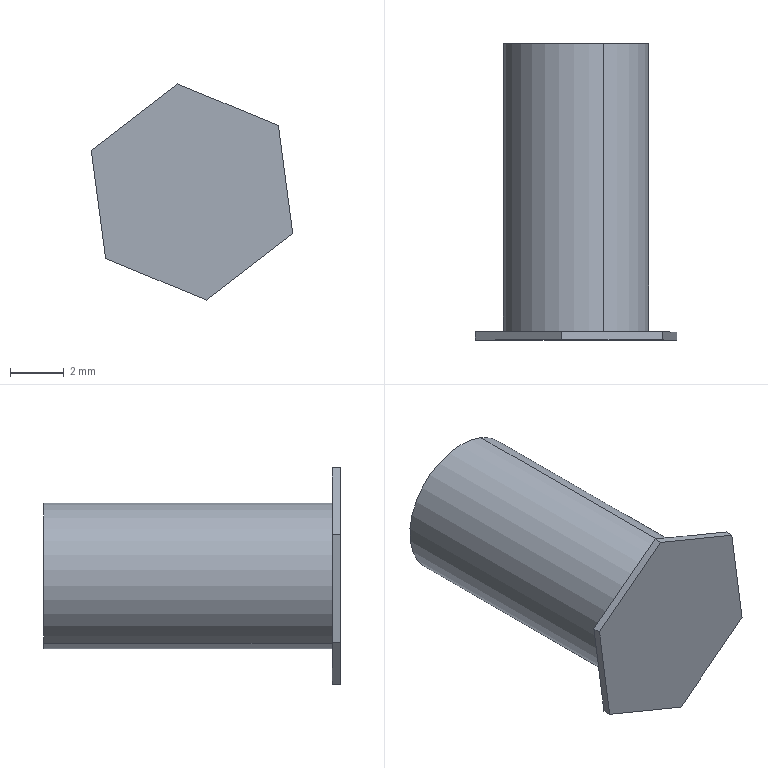Component | SolidWorks | P16BoxWeldment-1_BSO-M3-10-1 | 1 solid | 14 faces | box 7.48 x 11 x 8.02 mm | volume 201 mm3 | plane 10 | cylinder 4 | commonest cylinder face diameters 3 x2 5.4 x2
STEP:
#1=CARTESIAN_POINT('',(11.267,-9.398,0.4247));
#2=VERTEX_POINT('',#1);
#3=CARTESIAN_POINT('',(11.222,-9.398,0.3155));
#4=VERTEX_POINT('',#3);
#5=CARTESIAN_POINT('',(11.244,-9.398,0.3701));
#6=DIRECTION('',(-0.,1.,-0.));
#7=DIRECTION('',(-0.3816,0.,-0.9243));
#8=AXIS2_PLACEMENT_3D('',#5,#6,#7);
#9=CIRCLE('',#8,0.05906);
#10=EDGE_CURVE('',#2,#4,#9,.T.);
#11=ORIENTED_EDGE('',*,*,#10,.F.);
#12=CARTESIAN_POINT('',(11.267,-9.083,0.4247));
#13=VERTEX_POINT('',#12);
#14=CARTESIAN_POINT('',(11.267,-9.398,0.4247));
#15=DIRECTION('',(-0.,1.,-0.));
#16=VECTOR('',#15,39.37);
#17=LINE('',#14,#16);
#18=EDGE_CURVE('',#2,#13,#17,.T.);
#19=ORIENTED_EDGE('',*,*,#18,.T.);
#20=CARTESIAN_POINT('',(11.222,-9.083,0.3155));
#21=VERTEX_POINT('',#20);
#22=CARTESIAN_POINT('',(11.244,-9.083,0.3701));
#23=DIRECTION('',(-0.,1.,-0.));
#24=DIRECTION('',(-0.3816,0.,-0.9243));
#25=AXIS2_PLACEMENT_3D('',#22,#23,#24);
#26=CIRCLE('',#25,0.05906);
#27=EDGE_CURVE('',#13,#21,#26,.T.);
#28=ORIENTED_EDGE('',*,*,#27,.T.);
#29=CARTESIAN_POINT('',(11.222,-9.398,0.3155));
#30=DIRECTION('',(-0.,1.,-0.));
#31=VECTOR('',#30,39.37);
#32=LINE('',#29,#31);
#33=EDGE_CURVE('',#4,#21,#32,.T.);
#34=ORIENTED_EDGE('',*,*,#33,.F.);
#35=EDGE_LOOP('',(#11,#19,#28,#34));
#36=FACE_OUTER_BOUND('',#35,.T.);
#37=CARTESIAN_POINT('',(11.244,-9.398,0.3701));
#38=DIRECTION('',(-0.,1.,-0.));
#39=DIRECTION('',(-0.3816,0.,-0.9243));
#40=AXIS2_PLACEMENT_3D('',#37,#38,#39);
#41=CYLINDRICAL_SURFACE('',#40,0.05906);
#42=ADVANCED_FACE('',(#36),#41,.F.);
#43=CARTESIAN_POINT('',(11.204,-9.083,0.2718));
#44=VERTEX_POINT('',#43);
#45=CARTESIAN_POINT('',(11.285,-9.083,0.4683));
#46=VERTEX_POINT('',#45);
#47=CARTESIAN_POINT('',(11.244,-9.083,0.3701));
#48=DIRECTION('',(-0.,1.,-0.));
#49=DIRECTION('',(-0.3816,0.,-0.9243));
#50=AXIS2_PLACEMENT_3D('',#47,#48,#49);
#51=CIRCLE('',#50,0.1063);
#52=EDGE_CURVE('',#44,#46,#51,.T.);
#53=ORIENTED_EDGE('',*,*,#52,.F.);
#54=CARTESIAN_POINT('',(11.204,-9.504,0.2718));
#55=VERTEX_POINT('',#54);
#56=CARTESIAN_POINT('',(11.204,-9.083,0.2718));
#57=DIRECTION('',(0.,-1.,0.));
#58=VECTOR('',#57,39.37);
#59=LINE('',#56,#58);
#60=EDGE_CURVE('',#44,#55,#59,.T.);
#61=ORIENTED_EDGE('',*,*,#60,.T.);
#62=CARTESIAN_POINT('',(11.285,-9.504,0.4683));
#63=VERTEX_POINT('',#62);
#64=CARTESIAN_POINT('',(11.244,-9.504,0.3701));
#65=DIRECTION('',(0.,-1.,0.));
#66=DIRECTION('',(0.3816,0.,0.9243));
#67=AXIS2_PLACEMENT_3D('',#64,#65,#66);
#68=CIRCLE('',#67,0.1063);
#69=EDGE_CURVE('',#63,#55,#68,.T.);
#70=ORIENTED_EDGE('',*,*,#69,.F.);
#71=CARTESIAN_POINT('',(11.285,-9.083,0.4683));
#72=DIRECTION('',(0.,-1.,0.));
#73=VECTOR('',#72,39.37);
#74=LINE('',#71,#73);
#75=EDGE_CURVE('',#46,#63,#74,.T.);
#76=ORIENTED_EDGE('',*,*,#75,.F.);
#77=EDGE_LOOP('',(#53,#61,#70,#76));
#78=FACE_OUTER_BOUND('',#77,.T.);
#79=CARTESIAN_POINT('',(11.244,-9.083,0.3701));
#80=DIRECTION('',(0.,-1.,0.));
#81=DIRECTION('',(0.3816,0.,0.9243));
#82=AXIS2_PLACEMENT_3D('',#79,#80,#81);
#83=CYLINDRICAL_SURFACE('',#82,0.1063);
#84=ADVANCED_FACE('',(#78),#83,.T.);
#85=ORIENTED_EDGE('',*,*,#60,.F.);
#86=CARTESIAN_POINT('',(11.244,-9.083,0.3701));
#87=DIRECTION('',(-0.,1.,-0.));
#88=DIRECTION('',(-0.3816,0.,-0.9243));
#89=AXIS2_PLACEMENT_3D('',#86,#87,#88);
#90=CIRCLE('',#89,0.1063);
#91=EDGE_CURVE('',#46,#44,#90,.T.);
#92=ORIENTED_EDGE('',*,*,#91,.F.);
#93=ORIENTED_EDGE('',*,*,#75,.T.);
#94=CARTESIAN_POINT('',(11.244,-9.504,0.3701));
#95=DIRECTION('',(0.,-1.,0.));
#96=DIRECTION('',(0.3816,0.,0.9243));
#97=AXIS2_PLACEMENT_3D('',#94,#95,#96);
#98=CIRCLE('',#97,0.1063);
#99=EDGE_CURVE('',#55,#63,#98,.T.);
#100=ORIENTED_EDGE('',*,*,#99,.F.);
#101=EDGE_LOOP('',(#85,#92,#93,#100));
#102=FACE_OUTER_BOUND('',#101,.T.);
#103=CARTESIAN_POINT('',(11.244,-9.083,0.3701));
#104=DIRECTION('',(0.,-1.,0.));
#105=DIRECTION('',(0.3816,0.,0.9243));
#106=AXIS2_PLACEMENT_3D('',#103,#104,#105);
#107=CYLINDRICAL_SURFACE('',#106,0.1063);
#108=ADVANCED_FACE('',(#102),#107,.T.);
#109=CARTESIAN_POINT('',(11.244,-9.083,0.3701));
#110=DIRECTION('',(-0.,1.,-0.));
#111=DIRECTION('',(-0.3816,0.,-0.9243));
#112=AXIS2_PLACEMENT_3D('',#109,#110,#111);
#113=CIRCLE('',#112,0.05906);
#114=EDGE_CURVE('',#21,#13,#113,.T.);
#115=ORIENTED_EDGE('',*,*,#114,.F.);
#116=ORIENTED_EDGE('',*,*,#27,.F.);
#117=EDGE_LOOP('',(#115,#116));
#118=FACE_BOUND('',#117,.T.);
#119=ORIENTED_EDGE('',*,*,#91,.T.);
#120=ORIENTED_EDGE('',*,*,#52,.T.);
#121=EDGE_LOOP('',(#119,#120));
#122=FACE_OUTER_BOUND('',#121,.T.);
#123=CARTESIAN_POINT('',(11.244,-9.083,0.3701));
#124=DIRECTION('',(-0.,1.,-0.));
#125=DIRECTION('',(-0.3816,-0.,-0.9243));
#126=AXIS2_PLACEMENT_3D('',#123,#124,#125);
#127=PLANE('',#126);
#128=ADVANCED_FACE('',(#118,#122),#127,.T.);
#129=CARTESIAN_POINT('',(11.265,-9.504,0.2121));
#130=VERTEX_POINT('',#129);
#131=CARTESIAN_POINT('',(11.392,-9.504,0.3093));
#132=VERTEX_POINT('',#131);
#133=CARTESIAN_POINT('',(11.265,-9.504,0.2121));
#134=DIRECTION('',(0.7926,0.,0.6097));
#135=VECTOR('',#134,39.37);
#136=LINE('',#133,#135);
#137=EDGE_CURVE('',#130,#132,#136,.T.);
#138=ORIENTED_EDGE('',*,*,#137,.F.);
#139=CARTESIAN_POINT('',(11.118,-9.504,0.2729));
#140=VERTEX_POINT('',#139);
#141=CARTESIAN_POINT('',(11.118,-9.504,0.2729));
#142=DIRECTION('',(0.9243,-0.,-0.3816));
#143=VECTOR('',#142,39.37);
#144=LINE('',#141,#143);
#145=EDGE_CURVE('',#140,#130,#144,.T.);
#146=ORIENTED_EDGE('',*,*,#145,.F.);
#147=CARTESIAN_POINT('',(11.097,-9.504,0.4309));
#148=VERTEX_POINT('',#147);
#149=CARTESIAN_POINT('',(11.097,-9.504,0.4309));
#150=DIRECTION('',(0.1317,-0.,-0.9913));
#151=VECTOR('',#150,39.37);
#152=LINE('',#149,#151);
#153=EDGE_CURVE('',#148,#140,#152,.T.);
#154=ORIENTED_EDGE('',*,*,#153,.F.);
#155=CARTESIAN_POINT('',(11.223,-9.504,0.528));
#156=VERTEX_POINT('',#155);
#157=CARTESIAN_POINT('',(11.223,-9.504,0.528));
#158=DIRECTION('',(-0.7926,-0.,-0.6097));
#159=VECTOR('',#158,39.37);
#160=LINE('',#157,#159);
#161=EDGE_CURVE('',#156,#148,#160,.T.);
#162=ORIENTED_EDGE('',*,*,#161,.F.);
#163=CARTESIAN_POINT('',(11.371,-9.504,0.4672));
#164=VERTEX_POINT('',#163);
#165=CARTESIAN_POINT('',(11.371,-9.504,0.4672));
#166=DIRECTION('',(-0.9243,0.,0.3816));
#167=VECTOR('',#166,39.37);
#168=LINE('',#165,#167);
#169=EDGE_CURVE('',#164,#156,#168,.T.);
#170=ORIENTED_EDGE('',*,*,#169,.F.);
#171=CARTESIAN_POINT('',(11.392,-9.504,0.3093));
#172=DIRECTION('',(-0.1317,0.,0.9913));
#173=VECTOR('',#172,39.37);
#174=LINE('',#171,#173);
#175=EDGE_CURVE('',#132,#164,#174,.T.);
#176=ORIENTED_EDGE('',*,*,#175,.F.);
#177=EDGE_LOOP('',(#138,#146,#154,#162,#170,#176));
#178=FACE_OUTER_BOUND('',#177,.T.);
#179=ORIENTED_EDGE('',*,*,#69,.T.);
#180=ORIENTED_EDGE('',*,*,#99,.T.);
#181=EDGE_LOOP('',(#179,#180));
#182=FACE_BOUND('',#181,.T.);
#183=CARTESIAN_POINT('',(11.244,-9.504,0.3701));
#184=DIRECTION('',(0.,-1.,0.));
#185=DIRECTION('',(0.3816,0.,0.9243));
#186=AXIS2_PLACEMENT_3D('',#183,#184,#185);
#187=PLANE('',#186);
#188=ADVANCED_FACE('',(#178,#182),#187,.F.);
#189=CARTESIAN_POINT('',(11.265,-9.516,0.2121));
#190=VERTEX_POINT('',#189);
#191=CARTESIAN_POINT('',(11.392,-9.516,0.3093));
#192=VERTEX_POINT('',#191);
#193=CARTESIAN_POINT('',(11.265,-9.516,0.2121));
#194=DIRECTION('',(0.7926,0.,0.6097));
#195=VECTOR('',#194,39.37);
#196=LINE('',#193,#195);
#197=EDGE_CURVE('',#190,#192,#196,.T.);
#198=ORIENTED_EDGE('',*,*,#197,.F.);
#199=CARTESIAN_POINT('',(11.265,-9.504,0.2121));
#200=DIRECTION('',(0.,-1.,0.));
#201=VECTOR('',#200,39.37);
#202=LINE('',#199,#201);
#203=EDGE_CURVE('',#130,#190,#202,.T.);
#204=ORIENTED_EDGE('',*,*,#203,.F.);
#205=ORIENTED_EDGE('',*,*,#137,.T.);
#206=CARTESIAN_POINT('',(11.392,-9.504,0.3093));
#207=DIRECTION('',(0.,-1.,0.));
#208=VECTOR('',#207,39.37);
#209=LINE('',#206,#208);
#210=EDGE_CURVE('',#132,#192,#209,.T.);
#211=ORIENTED_EDGE('',*,*,#210,.T.);
#212=EDGE_LOOP('',(#198,#204,#205,#211));
#213=FACE_OUTER_BOUND('',#212,.T.);
#214=CARTESIAN_POINT('',(11.265,-9.504,0.2121));
#215=DIRECTION('',(0.6097,-0.,-0.7926));
#216=DIRECTION('',(-0.7926,-0.,-0.6097));
#217=AXIS2_PLACEMENT_3D('',#214,#215,#216);
#218=PLANE('',#217);
#219=ADVANCED_FACE('',(#213),#218,.T.);
#220=CARTESIAN_POINT('',(11.118,-9.516,0.2729));
#221=VERTEX_POINT('',#220);
#222=CARTESIAN_POINT('',(11.118,-9.516,0.2729));
#223=DIRECTION('',(0.9243,-0.,-0.3816));
#224=VECTOR('',#223,39.37);
#225=LINE('',#222,#224);
#226=EDGE_CURVE('',#221,#190,#225,.T.);
#227=ORIENTED_EDGE('',*,*,#226,.F.);
#228=CARTESIAN_POINT('',(11.118,-9.504,0.2729));
#229=DIRECTION('',(0.,-1.,0.));
#230=VECTOR('',#229,39.37);
#231=LINE('',#228,#230);
#232=EDGE_CURVE('',#140,#221,#231,.T.);
#233=ORIENTED_EDGE('',*,*,#232,.F.);
#234=ORIENTED_EDGE('',*,*,#145,.T.);
#235=ORIENTED_EDGE('',*,*,#203,.T.);
#236=EDGE_LOOP('',(#227,#233,#234,#235));
#237=FACE_OUTER_BOUND('',#236,.T.);
#238=CARTESIAN_POINT('',(11.118,-9.504,0.2729));
#239=DIRECTION('',(-0.3816,-0.,-0.9243));
#240=DIRECTION('',(-0.9243,0.,0.3816));
#241=AXIS2_PLACEMENT_3D('',#238,#239,#240);
#242=PLANE('',#241);
#243=ADVANCED_FACE('',(#237),#242,.T.);
#244=CARTESIAN_POINT('',(11.097,-9.516,0.4309));
#245=VERTEX_POINT('',#244);
#246=CARTESIAN_POINT('',(11.097,-9.516,0.4309));
#247=DIRECTION('',(0.1317,-0.,-0.9913));
#248=VECTOR('',#247,39.37);
#249=LINE('',#246,#248);
#250=EDGE_CURVE('',#245,#221,#249,.T.);
#251=ORIENTED_EDGE('',*,*,#250,.F.);
#252=CARTESIAN_POINT('',(11.097,-9.504,0.4309));
#253=DIRECTION('',(0.,-1.,0.));
#254=VECTOR('',#253,39.37);
#255=LINE('',#252,#254);
#256=EDGE_CURVE('',#148,#245,#255,.T.);
#257=ORIENTED_EDGE('',*,*,#256,.F.);
#258=ORIENTED_EDGE('',*,*,#153,.T.);
#259=ORIENTED_EDGE('',*,*,#232,.T.);
#260=EDGE_LOOP('',(#251,#257,#258,#259));
#261=FACE_OUTER_BOUND('',#260,.T.);
#262=CARTESIAN_POINT('',(11.097,-9.504,0.4309));
#263=DIRECTION('',(-0.9913,-0.,-0.1317));
#264=DIRECTION('',(-0.1317,0.,0.9913));
#265=AXIS2_PLACEMENT_3D('',#262,#263,#264);
#266=PLANE('',#265);
#267=ADVANCED_FACE('',(#261),#266,.T.);
#268=CARTESIAN_POINT('',(11.223,-9.516,0.528));
#269=VERTEX_POINT('',#268);
#270=CARTESIAN_POINT('',(11.223,-9.516,0.528));
#271=DIRECTION('',(-0.7926,-0.,-0.6097));
#272=VECTOR('',#271,39.37);
#273=LINE('',#270,#272);
#274=EDGE_CURVE('',#269,#245,#273,.T.);
#275=ORIENTED_EDGE('',*,*,#274,.F.);
#276=CARTESIAN_POINT('',(11.223,-9.504,0.528));
#277=DIRECTION('',(0.,-1.,0.));
#278=VECTOR('',#277,39.37);
#279=LINE('',#276,#278);
#280=EDGE_CURVE('',#156,#269,#279,.T.);
#281=ORIENTED_EDGE('',*,*,#280,.F.);
#282=ORIENTED_EDGE('',*,*,#161,.T.);
#283=ORIENTED_EDGE('',*,*,#256,.T.);
#284=EDGE_LOOP('',(#275,#281,#282,#283));
#285=FACE_OUTER_BOUND('',#284,.T.);
#286=CARTESIAN_POINT('',(11.223,-9.504,0.528));
#287=DIRECTION('',(-0.6097,0.,0.7926));
#288=DIRECTION('',(0.7926,0.,0.6097));
#289=AXIS2_PLACEMENT_3D('',#286,#287,#288);
#290=PLANE('',#289);
#291=ADVANCED_FACE('',(#285),#290,.T.);
#292=CARTESIAN_POINT('',(11.371,-9.516,0.4672));
#293=VERTEX_POINT('',#292);
#294=CARTESIAN_POINT('',(11.371,-9.516,0.4672));
#295=DIRECTION('',(-0.9243,0.,0.3816));
#296=VECTOR('',#295,39.37);
#297=LINE('',#294,#296);
#298=EDGE_CURVE('',#293,#269,#297,.T.);
#299=ORIENTED_EDGE('',*,*,#298,.F.);
#300=CARTESIAN_POINT('',(11.371,-9.504,0.4672));
#301=DIRECTION('',(0.,-1.,0.));
#302=VECTOR('',#301,39.37);
#303=LINE('',#300,#302);
#304=EDGE_CURVE('',#164,#293,#303,.T.);
#305=ORIENTED_EDGE('',*,*,#304,.F.);
#306=ORIENTED_EDGE('',*,*,#169,.T.);
#307=ORIENTED_EDGE('',*,*,#280,.T.);
#308=EDGE_LOOP('',(#299,#305,#306,#307));
#309=FACE_OUTER_BOUND('',#308,.T.);
#310=CARTESIAN_POINT('',(11.371,-9.504,0.4672));
#311=DIRECTION('',(0.3816,0.,0.9243));
#312=DIRECTION('',(0.9243,-0.,-0.3816));
#313=AXIS2_PLACEMENT_3D('',#310,#311,#312);
#314=PLANE('',#313);
#315=ADVANCED_FACE('',(#309),#314,.T.);
#316=CARTESIAN_POINT('',(11.392,-9.516,0.3093));
#317=DIRECTION('',(-0.1317,0.,0.9913));
#318=VECTOR('',#317,39.37);
#319=LINE('',#316,#318);
#320=EDGE_CURVE('',#192,#293,#319,.T.);
#321=ORIENTED_EDGE('',*,*,#320,.F.);
#322=ORIENTED_EDGE('',*,*,#210,.F.);
#323=ORIENTED_EDGE('',*,*,#175,.T.);
#324=ORIENTED_EDGE('',*,*,#304,.T.);
#325=EDGE_LOOP('',(#321,#322,#323,#324));
#326=FACE_OUTER_BOUND('',#325,.T.);
#327=CARTESIAN_POINT('',(11.392,-9.504,0.3093));
#328=DIRECTION('',(0.9913,0.,0.1317));
#329=DIRECTION('',(0.1317,-0.,-0.9913));
#330=AXIS2_PLACEMENT_3D('',#327,#328,#329);
#331=PLANE('',#330);
#332=ADVANCED_FACE('',(#326),#331,.T.);
#333=ORIENTED_EDGE('',*,*,#197,.T.);
#334=ORIENTED_EDGE('',*,*,#320,.T.);
#335=ORIENTED_EDGE('',*,*,#298,.T.);
#336=ORIENTED_EDGE('',*,*,#274,.T.);
#337=ORIENTED_EDGE('',*,*,#250,.T.);
#338=ORIENTED_EDGE('',*,*,#226,.T.);
#339=EDGE_LOOP('',(#333,#334,#335,#336,#337,#338));
#340=FACE_OUTER_BOUND('',#339,.T.);
#341=CARTESIAN_POINT('',(11.244,-9.516,0.3701));
#342=DIRECTION('',(-0.,1.,-0.));
#343=DIRECTION('',(-0.3816,-0.,-0.9243));
#344=AXIS2_PLACEMENT_3D('',#341,#342,#343);
#345=PLANE('',#344);
#346=ADVANCED_FACE('',(#340),#345,.F.);
#347=ORIENTED_EDGE('',*,*,#18,.F.);
#348=CARTESIAN_POINT('',(11.244,-9.398,0.3701));
#349=DIRECTION('',(-0.,1.,-0.));
#350=DIRECTION('',(-0.3816,0.,-0.9243));
#351=AXIS2_PLACEMENT_3D('',#348,#349,#350);
#352=CIRCLE('',#351,0.05906);
#353=EDGE_CURVE('',#4,#2,#352,.T.);
#354=ORIENTED_EDGE('',*,*,#353,.F.);
#355=ORIENTED_EDGE('',*,*,#33,.T.);
#356=ORIENTED_EDGE('',*,*,#114,.T.);
#357=EDGE_LOOP('',(#347,#354,#355,#356));
#358=FACE_OUTER_BOUND('',#357,.T.);
#359=CARTESIAN_POINT('',(11.244,-9.398,0.3701));
#360=DIRECTION('',(-0.,1.,-0.));
#361=DIRECTION('',(-0.3816,0.,-0.9243));
#362=AXIS2_PLACEMENT_3D('',#359,#360,#361);
#363=CYLINDRICAL_SURFACE('',#362,0.05906);
#364=ADVANCED_FACE('',(#358),#363,.F.);
#365=ORIENTED_EDGE('',*,*,#353,.T.);
#366=ORIENTED_EDGE('',*,*,#10,.T.);
#367=EDGE_LOOP('',(#365,#366));
#368=FACE_OUTER_BOUND('',#367,.T.);
#369=CARTESIAN_POINT('',(11.244,-9.398,0.3701));
#370=DIRECTION('',(-0.,1.,-0.));
#371=DIRECTION('',(-0.3816,-0.,-0.9243));
#372=AXIS2_PLACEMENT_3D('',#369,#370,#371);
#373=PLANE('',#372);
#374=ADVANCED_FACE('',(#368),#373,.T.);
#375=CLOSED_SHELL('',(#42,#84,#108,#128,#188,#219,#243,#267,#291,#315,#332,#346,#364,#374));
#376=MANIFOLD_SOLID_BREP('',#375);
#377=CARTESIAN_POINT('',(0.,0.,0.));
#378=DIRECTION('',(0.,0.,1.));
#379=DIRECTION('',(1.,0.,0.));
#380=AXIS2_PLACEMENT_3D('',#377,#378,#379);
#381=(LENGTH_UNIT()NAMED_UNIT(*)SI_UNIT($,.METRE.));
#382=LENGTH_MEASURE_WITH_UNIT(LENGTH_MEASURE(0.0254),#381);
#383=DIMENSIONAL_EXPONENTS(1.,0.,0.,0.,0.,0.,0.);
#384=(CONVERSION_BASED_UNIT('',#382)LENGTH_UNIT()NAMED_UNIT(#383));
#385=UNCERTAINTY_MEASURE_WITH_UNIT(LENGTH_MEASURE(0.00001),#384,'','');
#386=(NAMED_UNIT(*)PLANE_ANGLE_UNIT()SI_UNIT($,.RADIAN.));
#387=(NAMED_UNIT(*)SI_UNIT($,.STERADIAN.)SOLID_ANGLE_UNIT());
#388=(GEOMETRIC_REPRESENTATION_CONTEXT(3)GLOBAL_UNCERTAINTY_ASSIGNED_CONTEXT((#385))GLOBAL_UNIT_ASSIGNED_CONTEXT((#384,#386,#387))REPRESENTATION_CONTEXT('',''));
#389=ADVANCED_BREP_SHAPE_REPRESENTATION('',(#376,#380),#388);
#390=COLOUR_RGB('',0.7922,0.8196,0.9333);
#391=FILL_AREA_STYLE_COLOUR('',#390);
#392=FILL_AREA_STYLE('',(#391));
#393=SURFACE_STYLE_FILL_AREA(#392);
#394=SURFACE_SIDE_STYLE('',(#393));
#395=SURFACE_STYLE_USAGE(.BOTH.,#394);
#396=PRESENTATION_STYLE_ASSIGNMENT((#395));
#397=STYLED_ITEM('',(#396),#376);
#398=(LENGTH_UNIT()NAMED_UNIT(*)SI_UNIT($,.METRE.));
#399=LENGTH_MEASURE_WITH_UNIT(LENGTH_MEASURE(0.0254),#398);
#400=DIMENSIONAL_EXPONENTS(1.,0.,0.,0.,0.,0.,0.);
#401=(CONVERSION_BASED_UNIT('',#399)LENGTH_UNIT()NAMED_UNIT(#400));
#402=UNCERTAINTY_MEASURE_WITH_UNIT(LENGTH_MEASURE(0.00001),#401,'','');
#403=(NAMED_UNIT(*)PLANE_ANGLE_UNIT()SI_UNIT($,.RADIAN.));
#404=(NAMED_UNIT(*)SI_UNIT($,.STERADIAN.)SOLID_ANGLE_UNIT());
#405=(GEOMETRIC_REPRESENTATION_CONTEXT(3)GLOBAL_UNCERTAINTY_ASSIGNED_CONTEXT((#402))GLOBAL_UNIT_ASSIGNED_CONTEXT((#401,#403,#404))REPRESENTATION_CONTEXT('',''));
#406=MECHANICAL_DESIGN_GEOMETRIC_PRESENTATION_REPRESENTATION('',(#397),#405);
#407=PRESENTATION_LAYER_ASSIGNMENT('','',(#397));